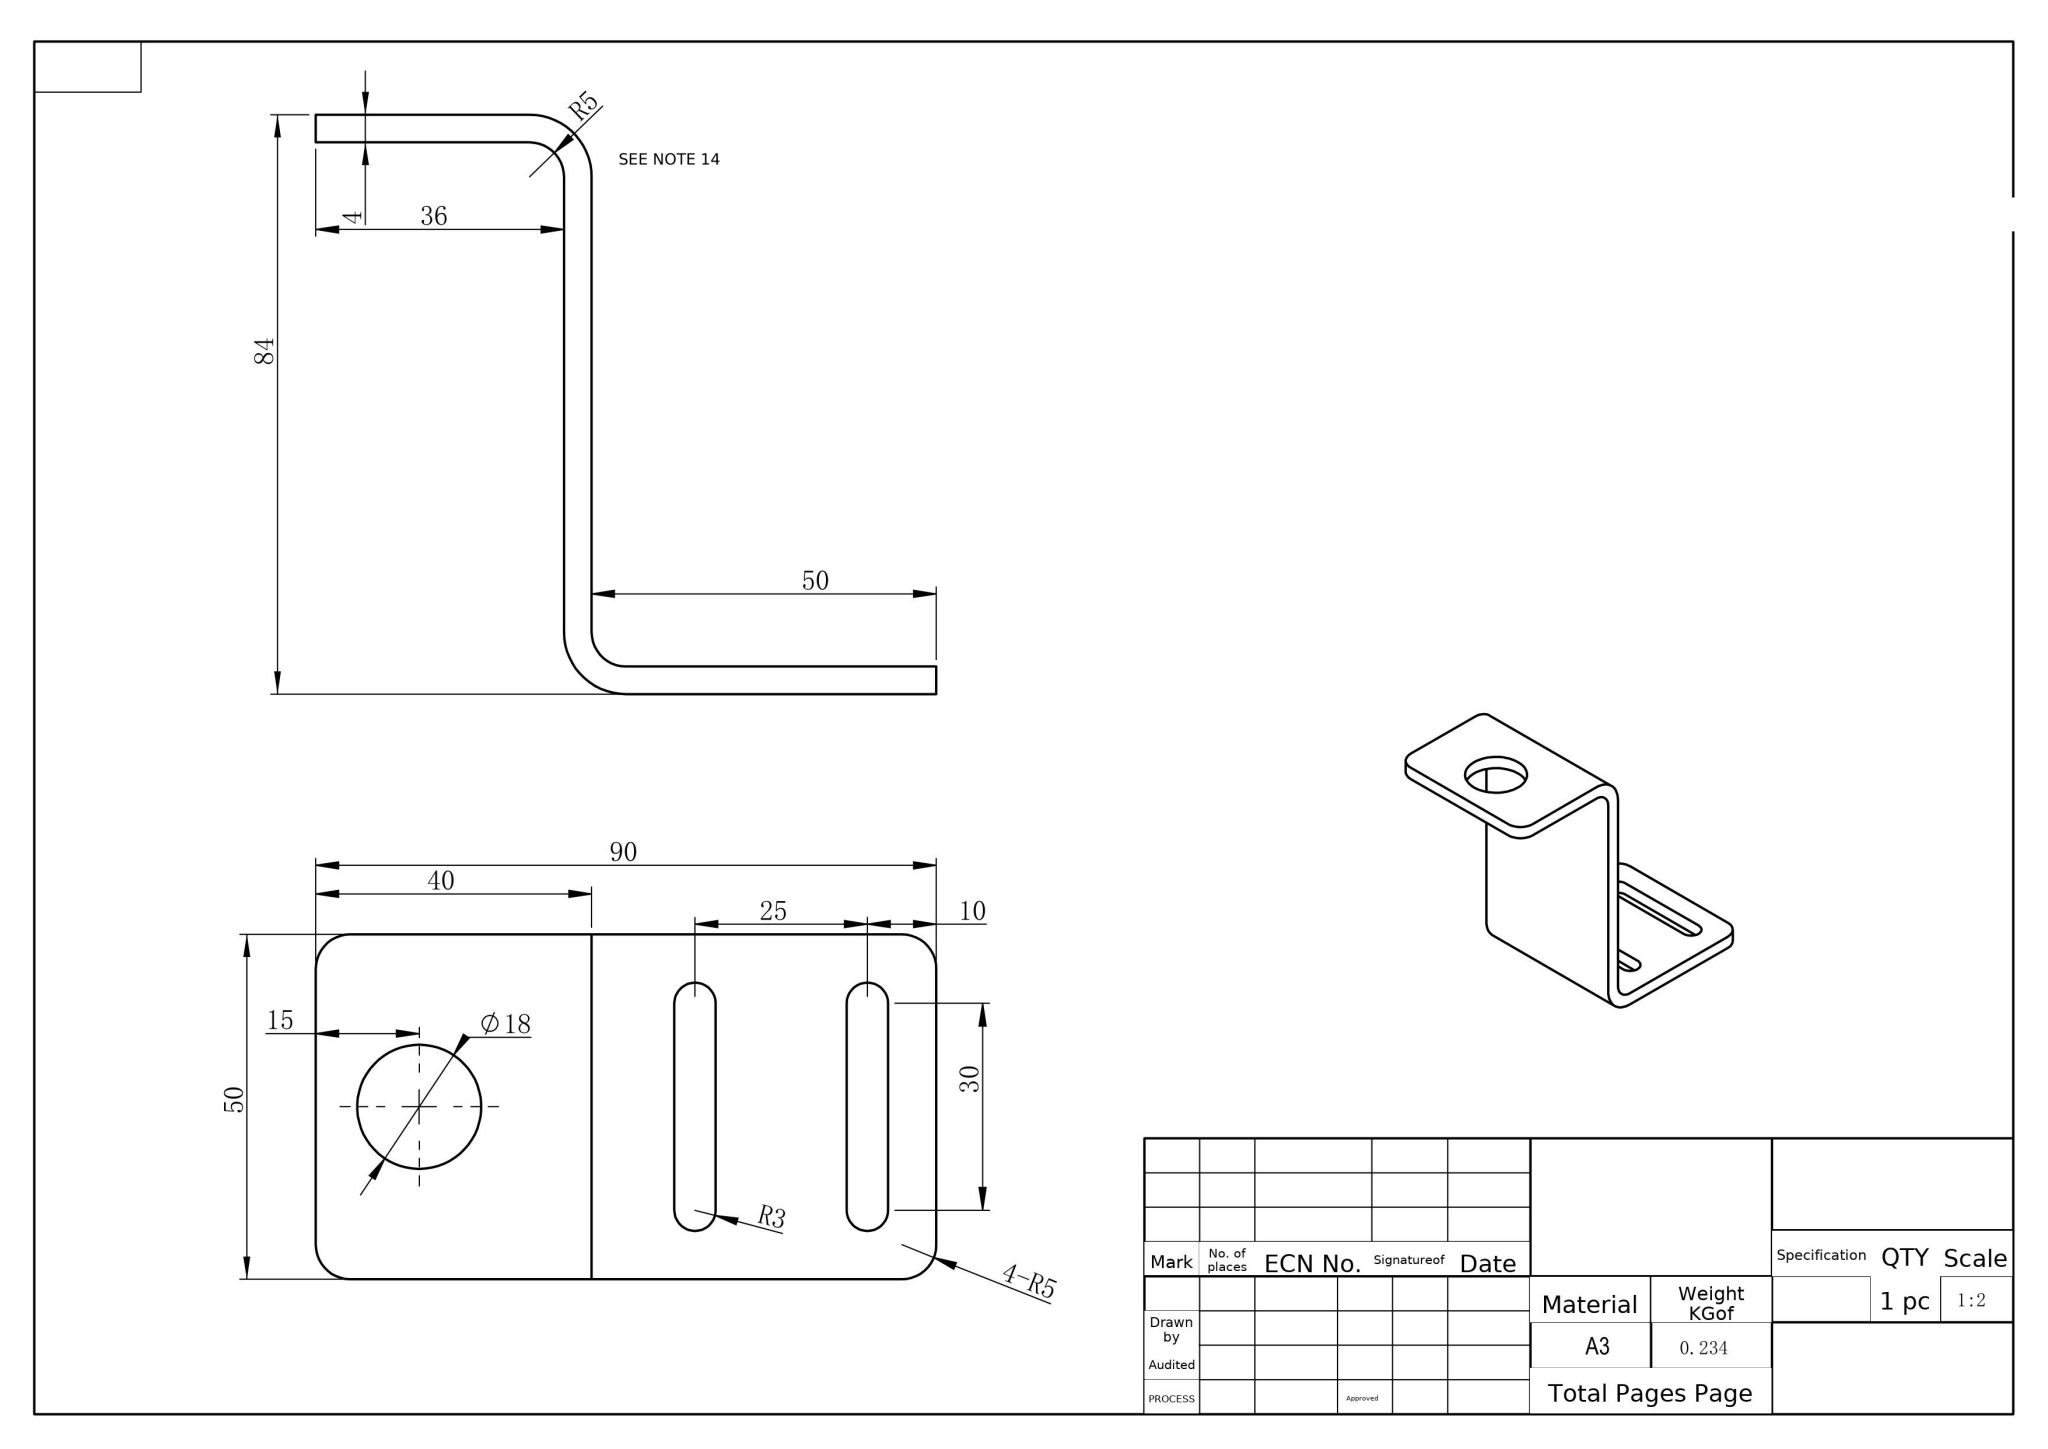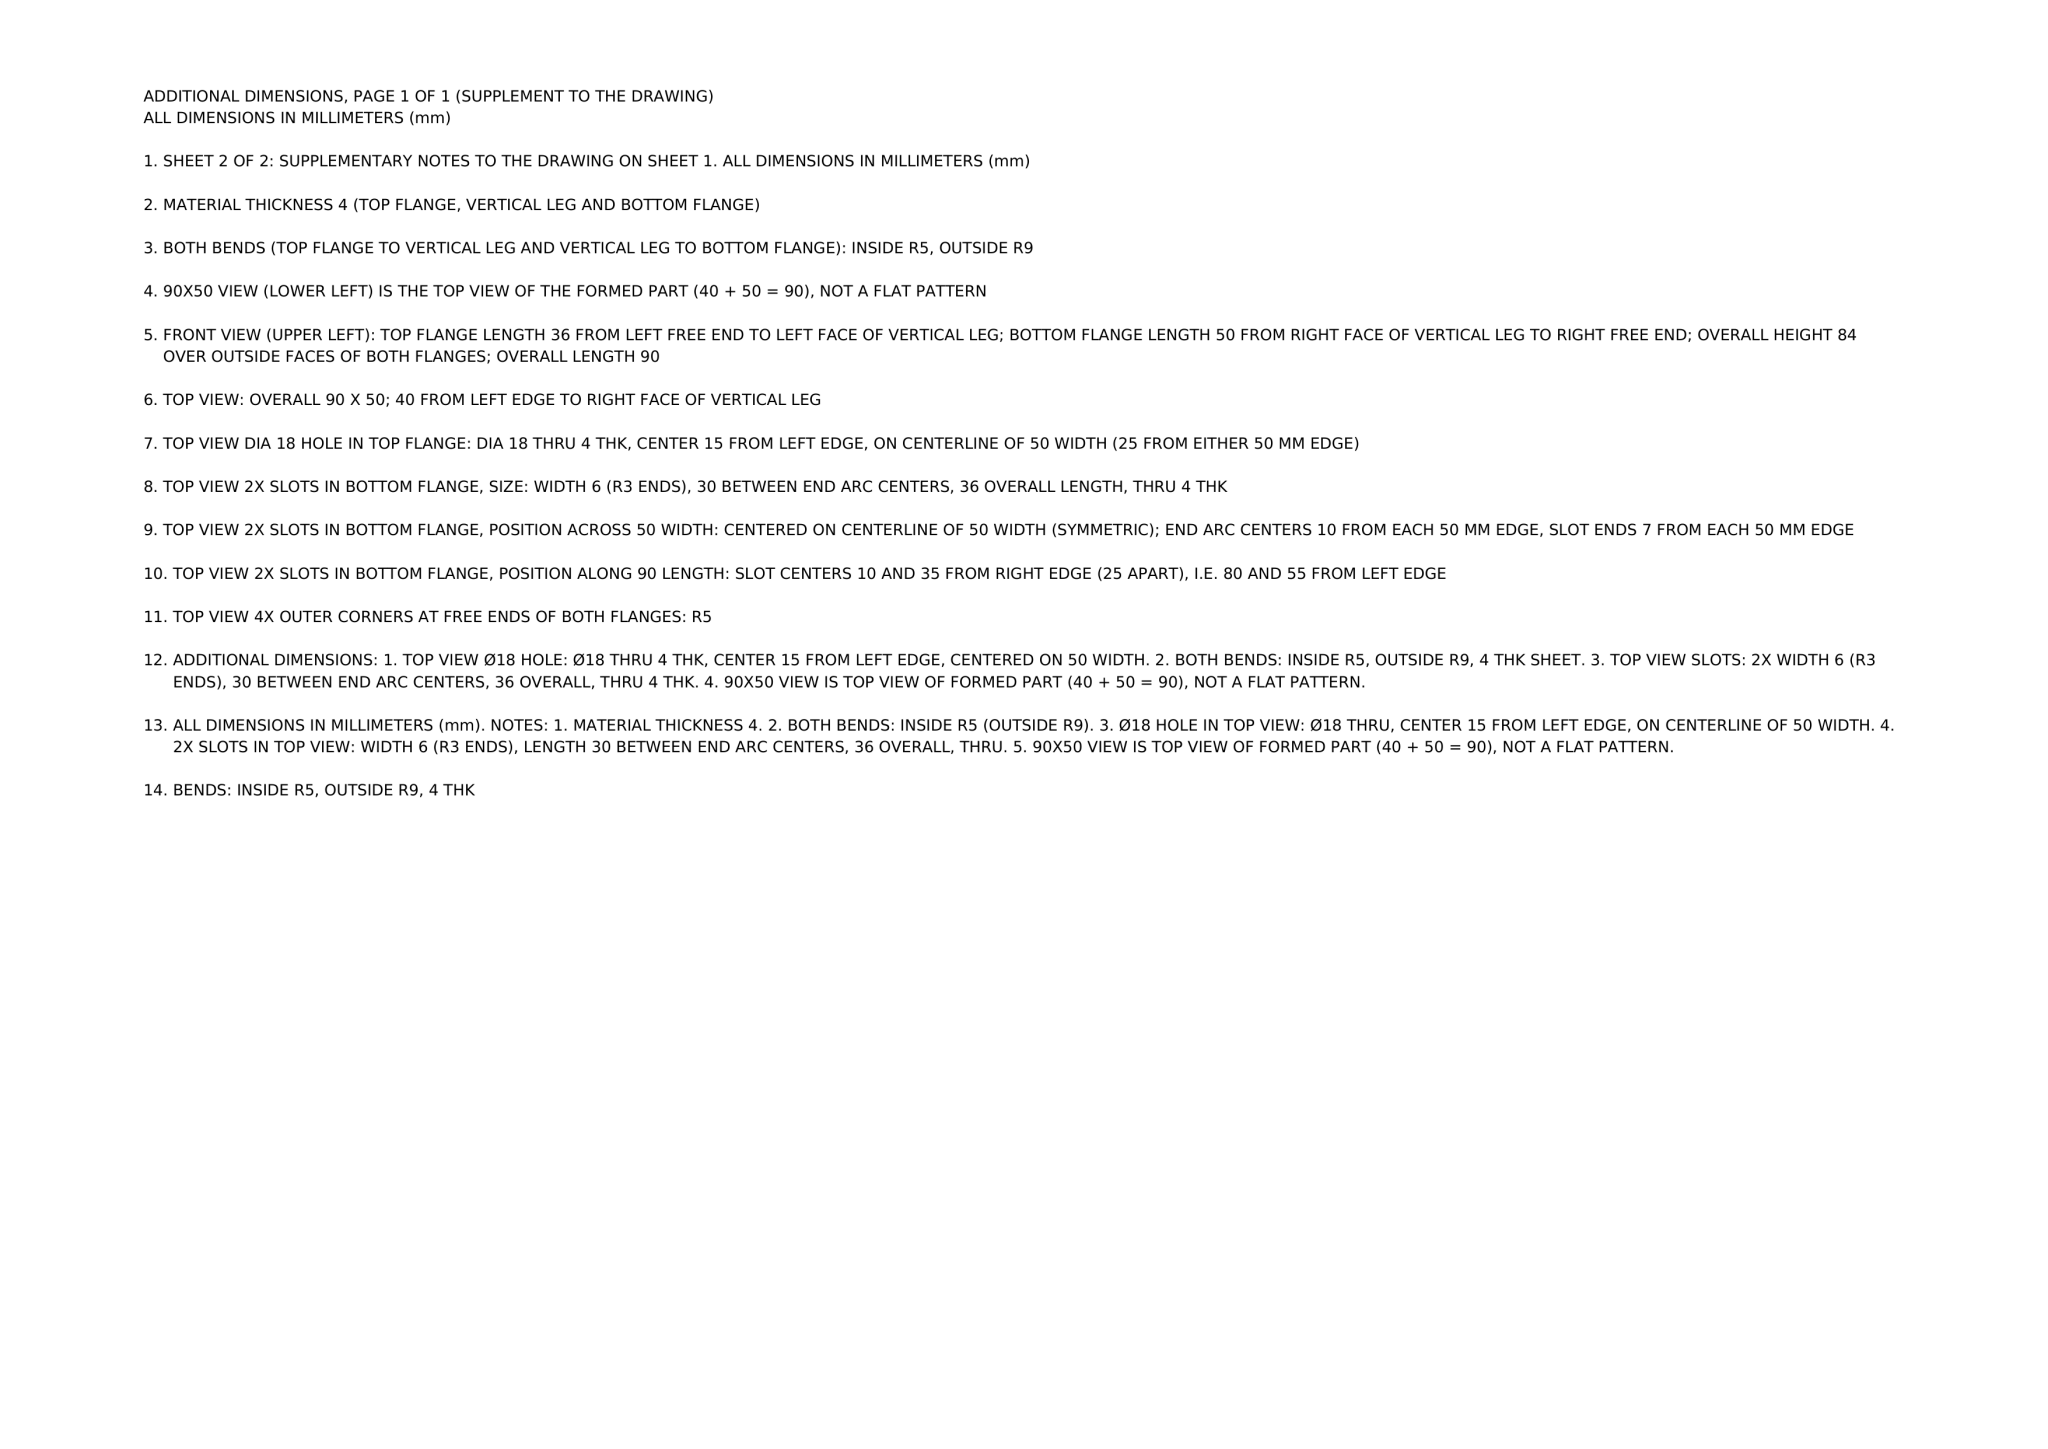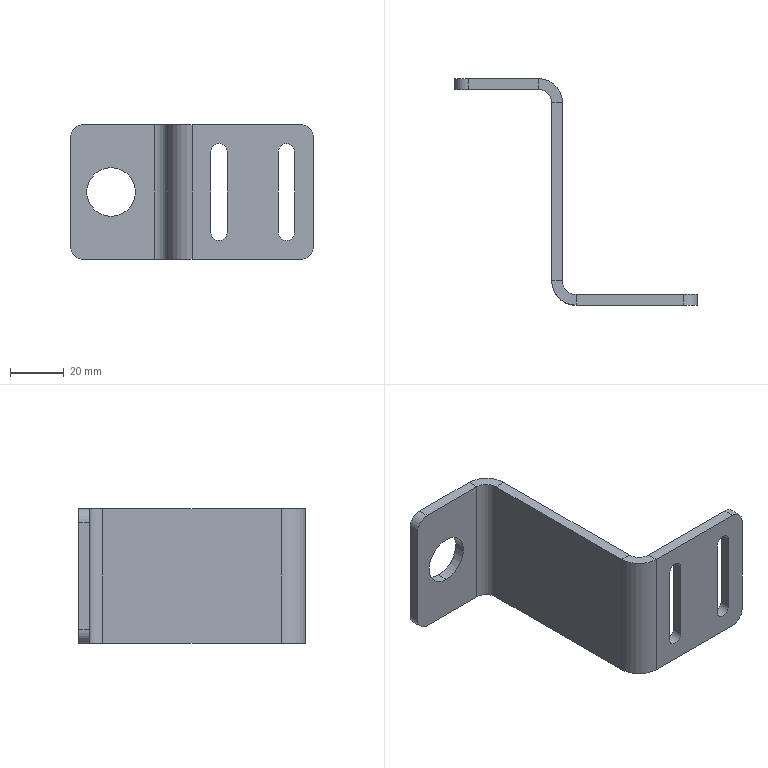Part | NX | mm | 1 solid | 38 faces | box 90 x 84 x 50 mm | volume 30028 mm3 | plane 22 | cylinder 16 | commonest cylinder face diameters 6 x6 10 x6 18 x4